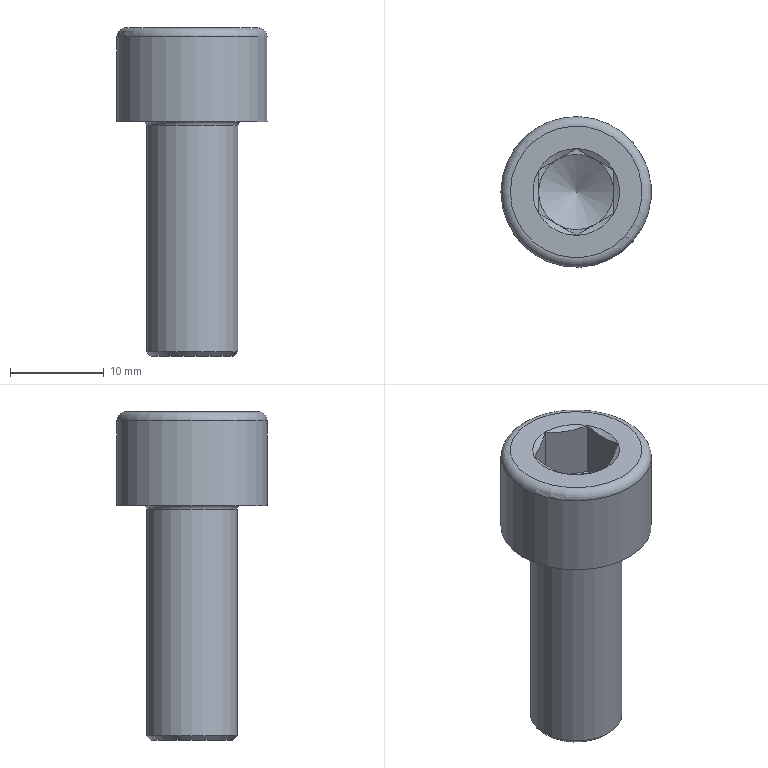Component | NX | GB-T70_1-2000_M10X25_2 | 1 solid | 27 faces | volume 3484 mm3 | plane 15 | cone 8 | cylinder 2 | torus 2 | commonest cylinder face diameters 9.732 x1 16 x1